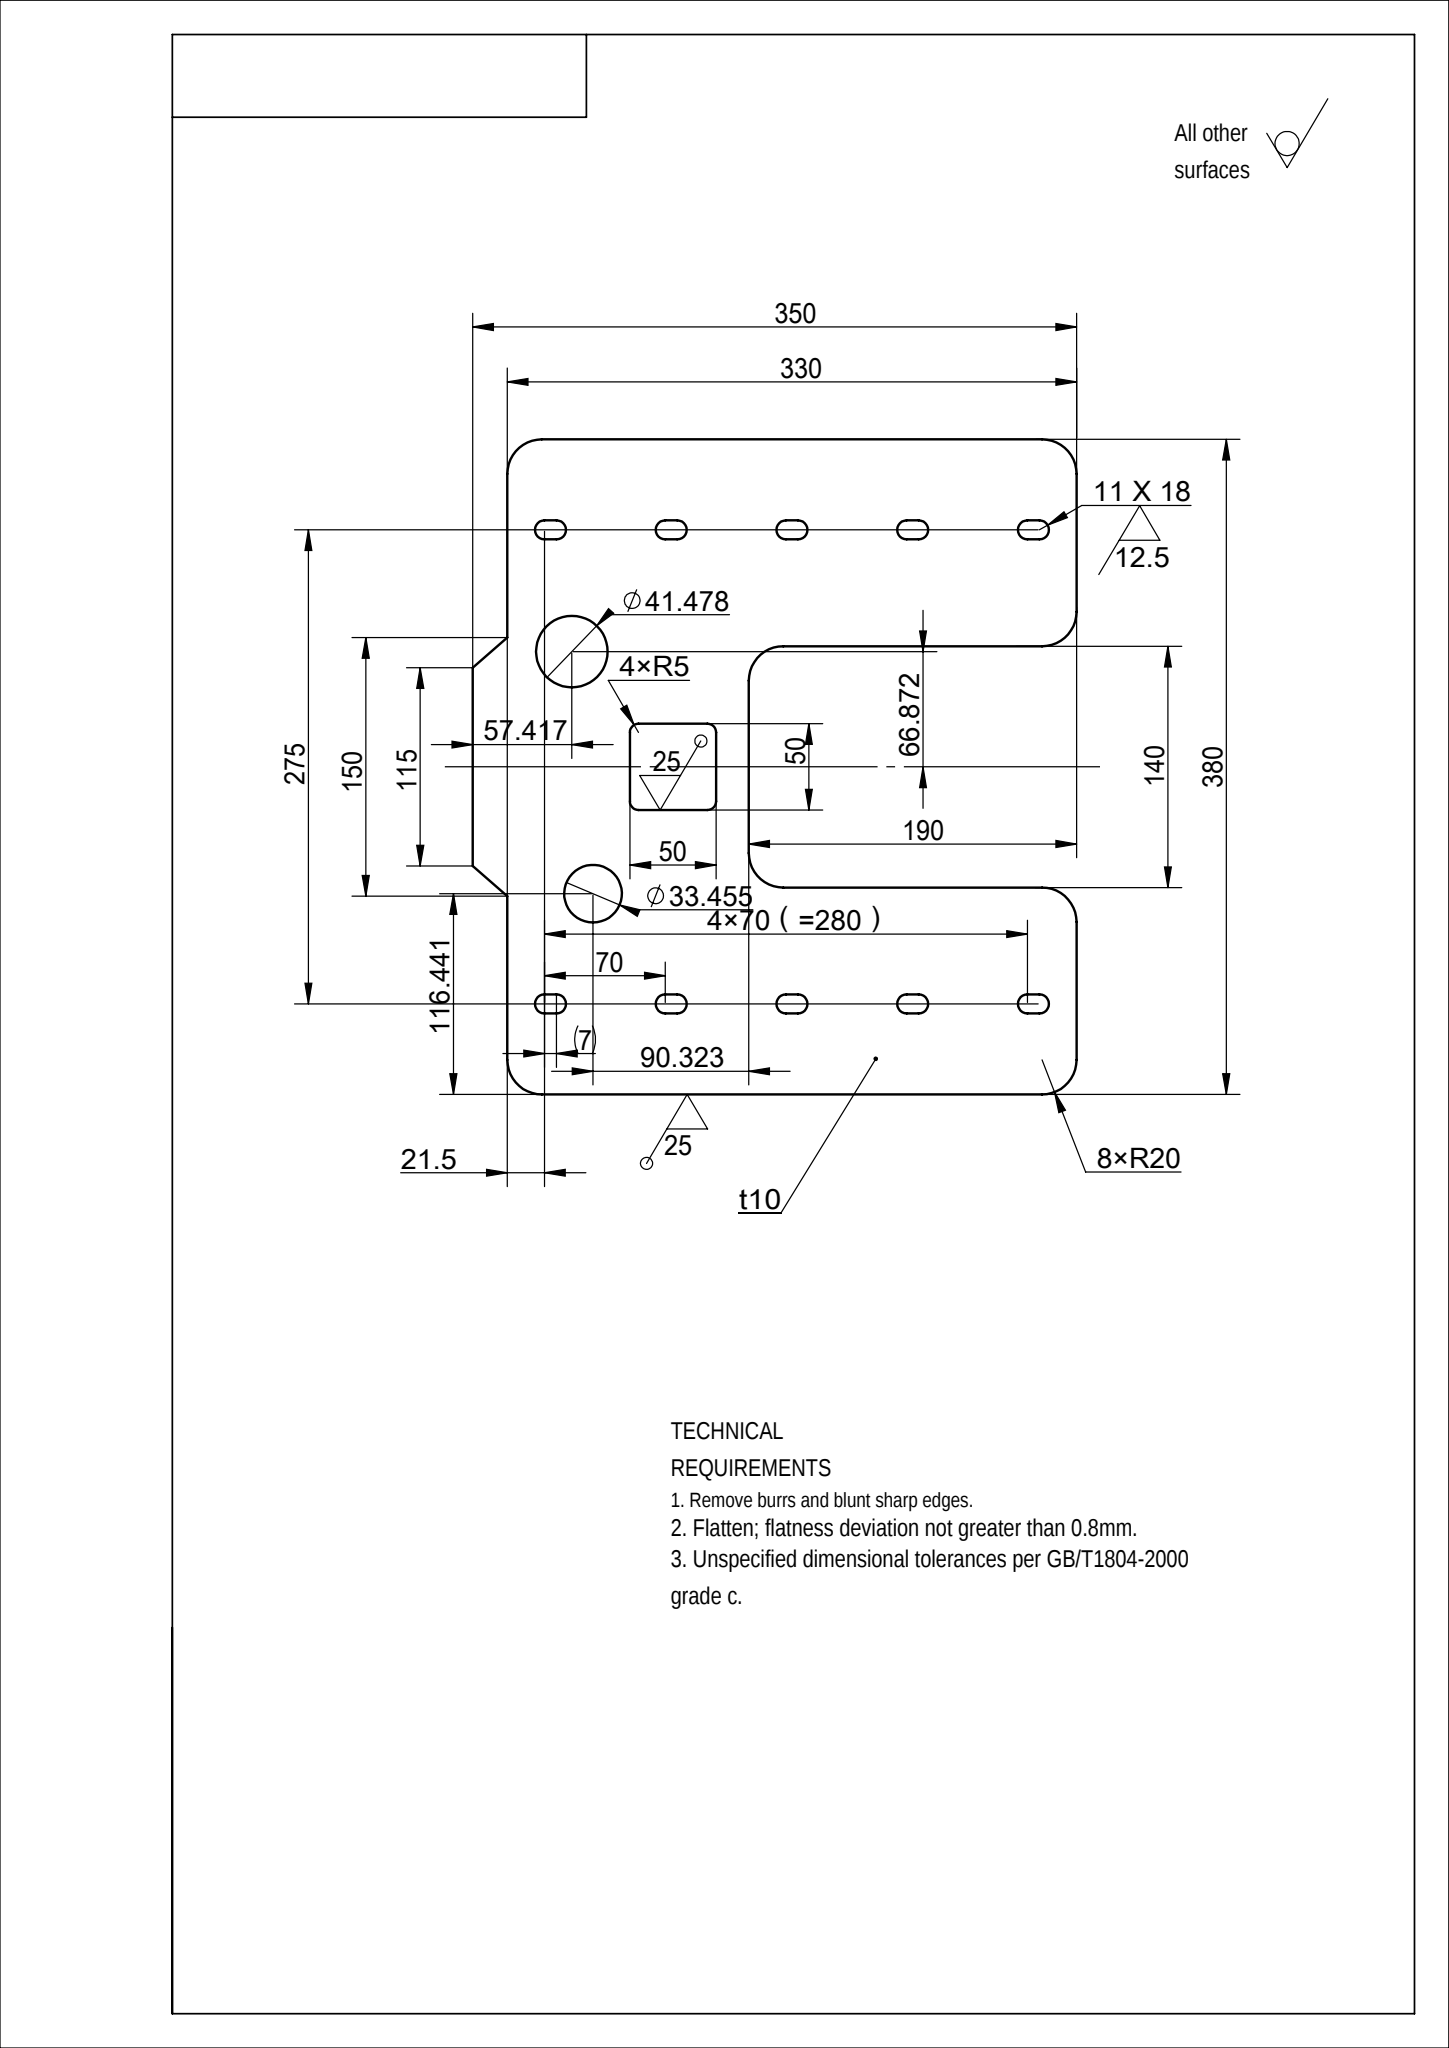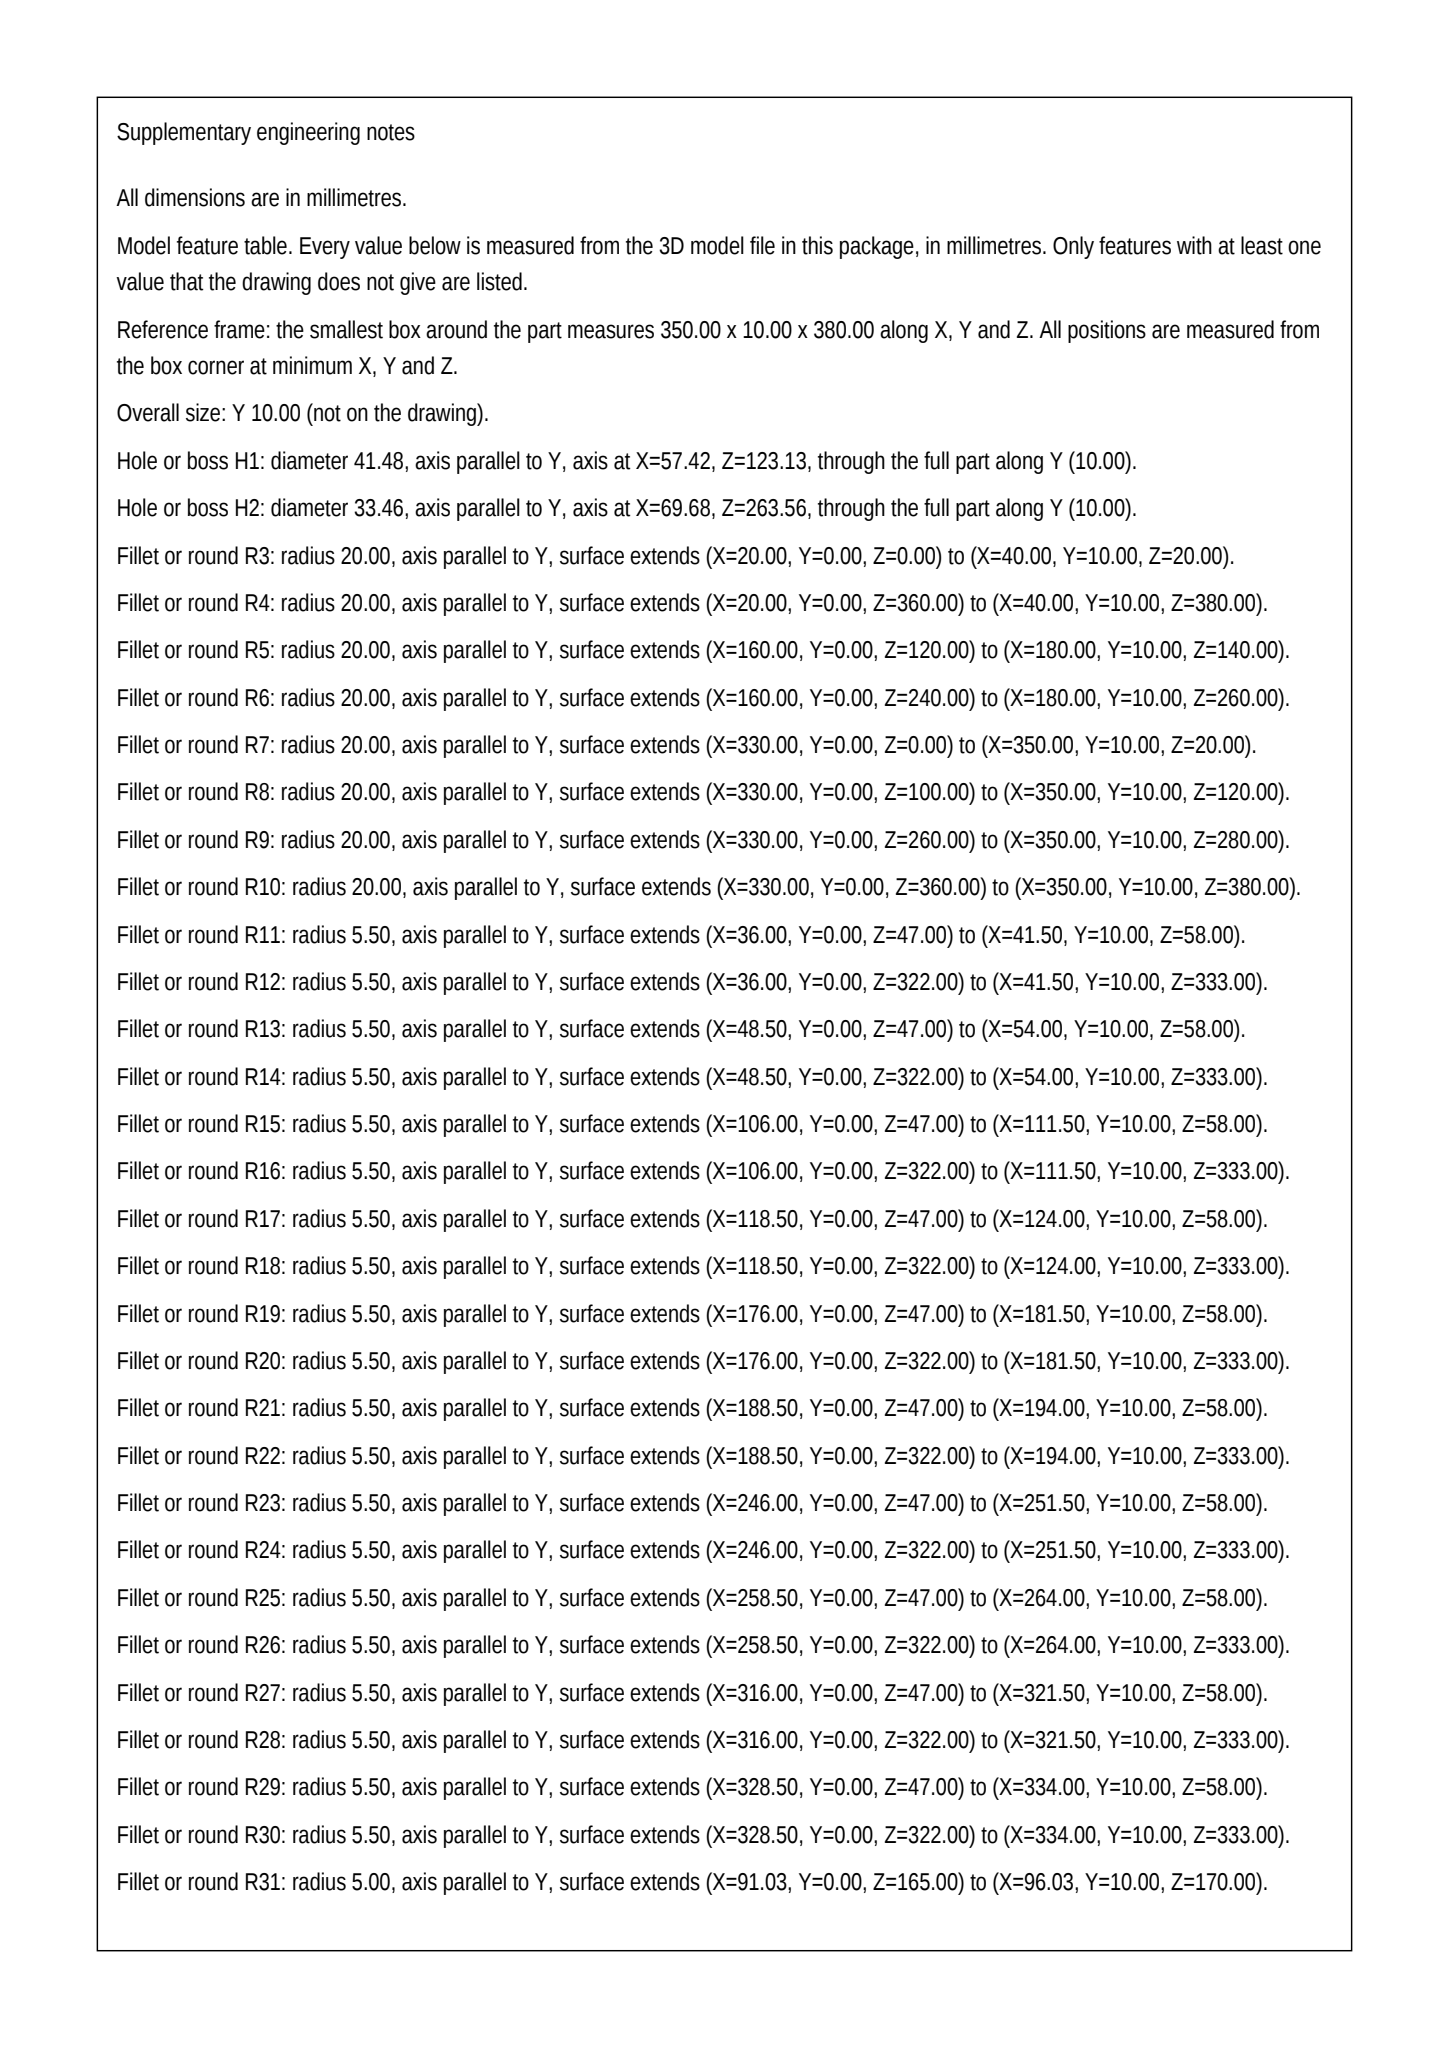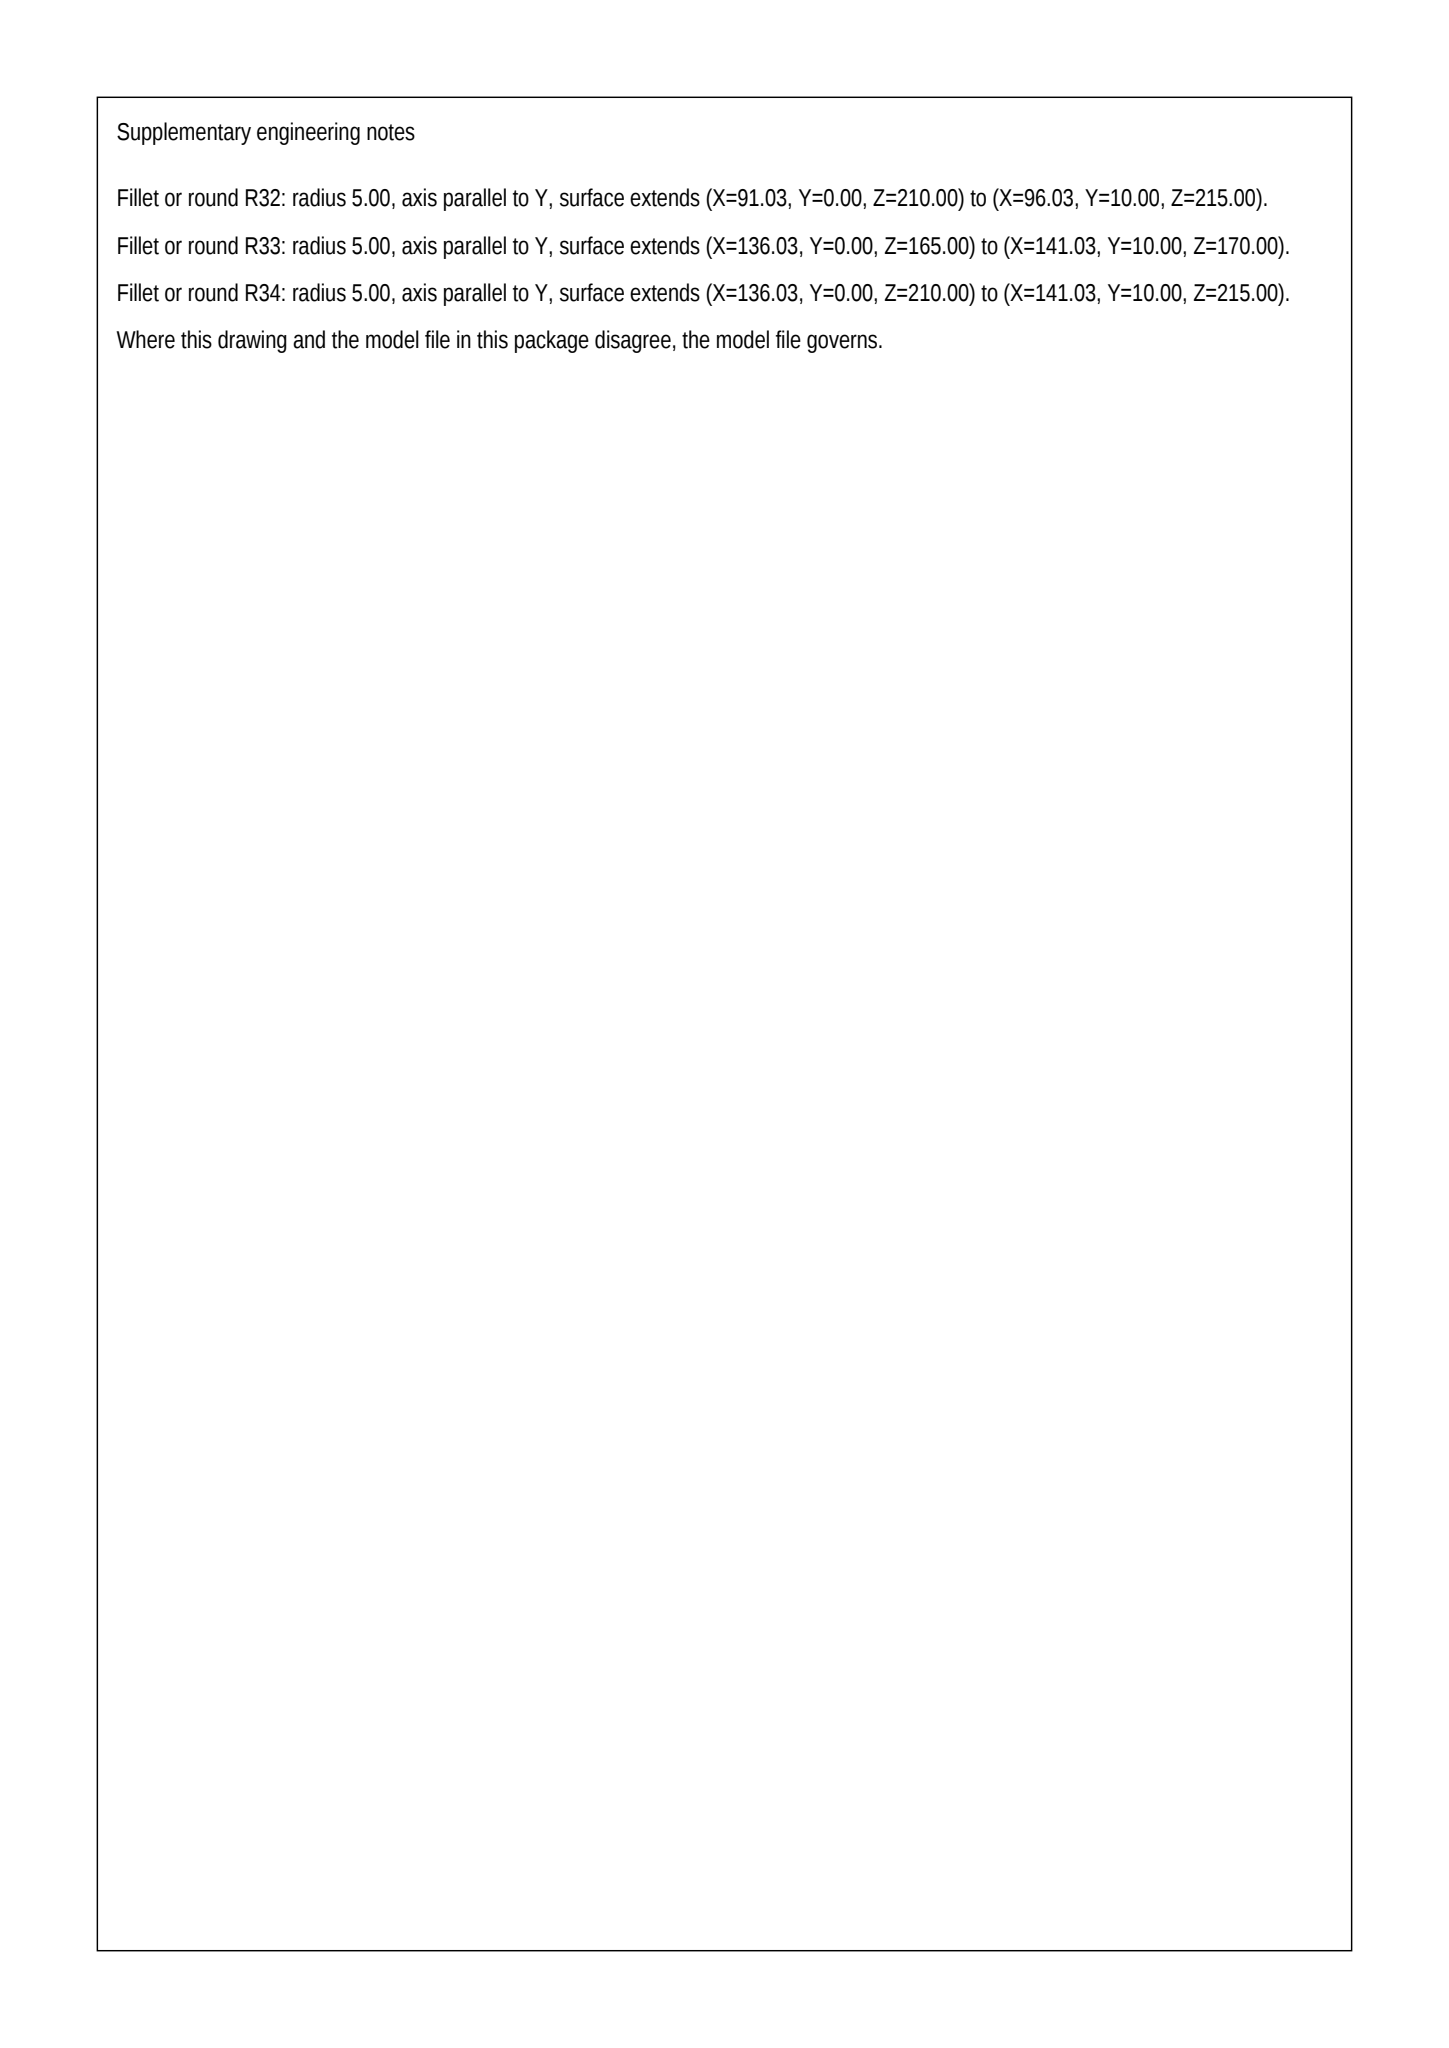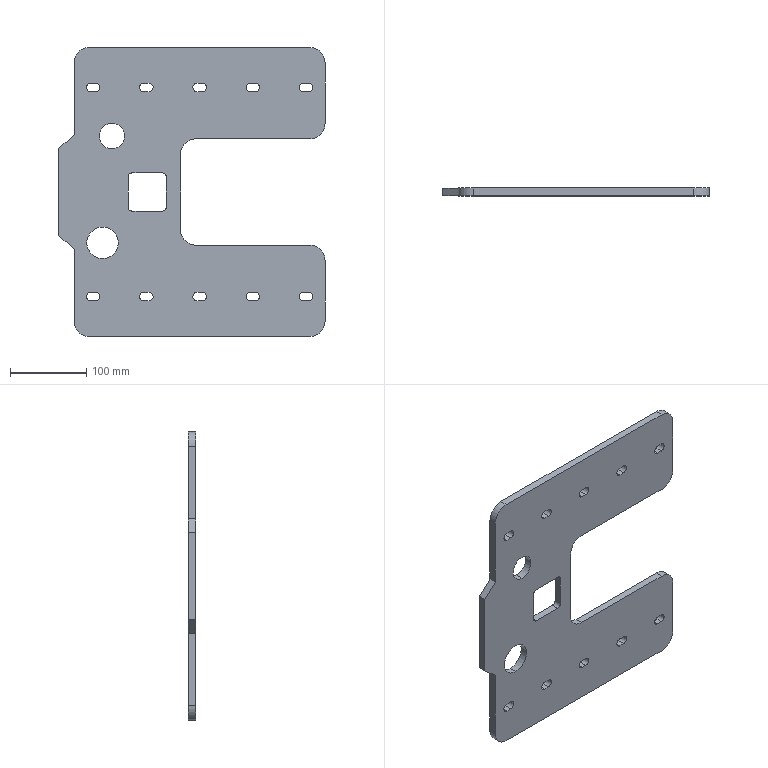Part | SolidWorks | mm | 1 solid | 74 faces | box 350 x 10 x 380 mm | volume 946775 mm3 | plane 38 | cylinder 36 | commonest cylinder face diameters 11 x20 40 x8 10 x4 41.478 x2 33.455 x2